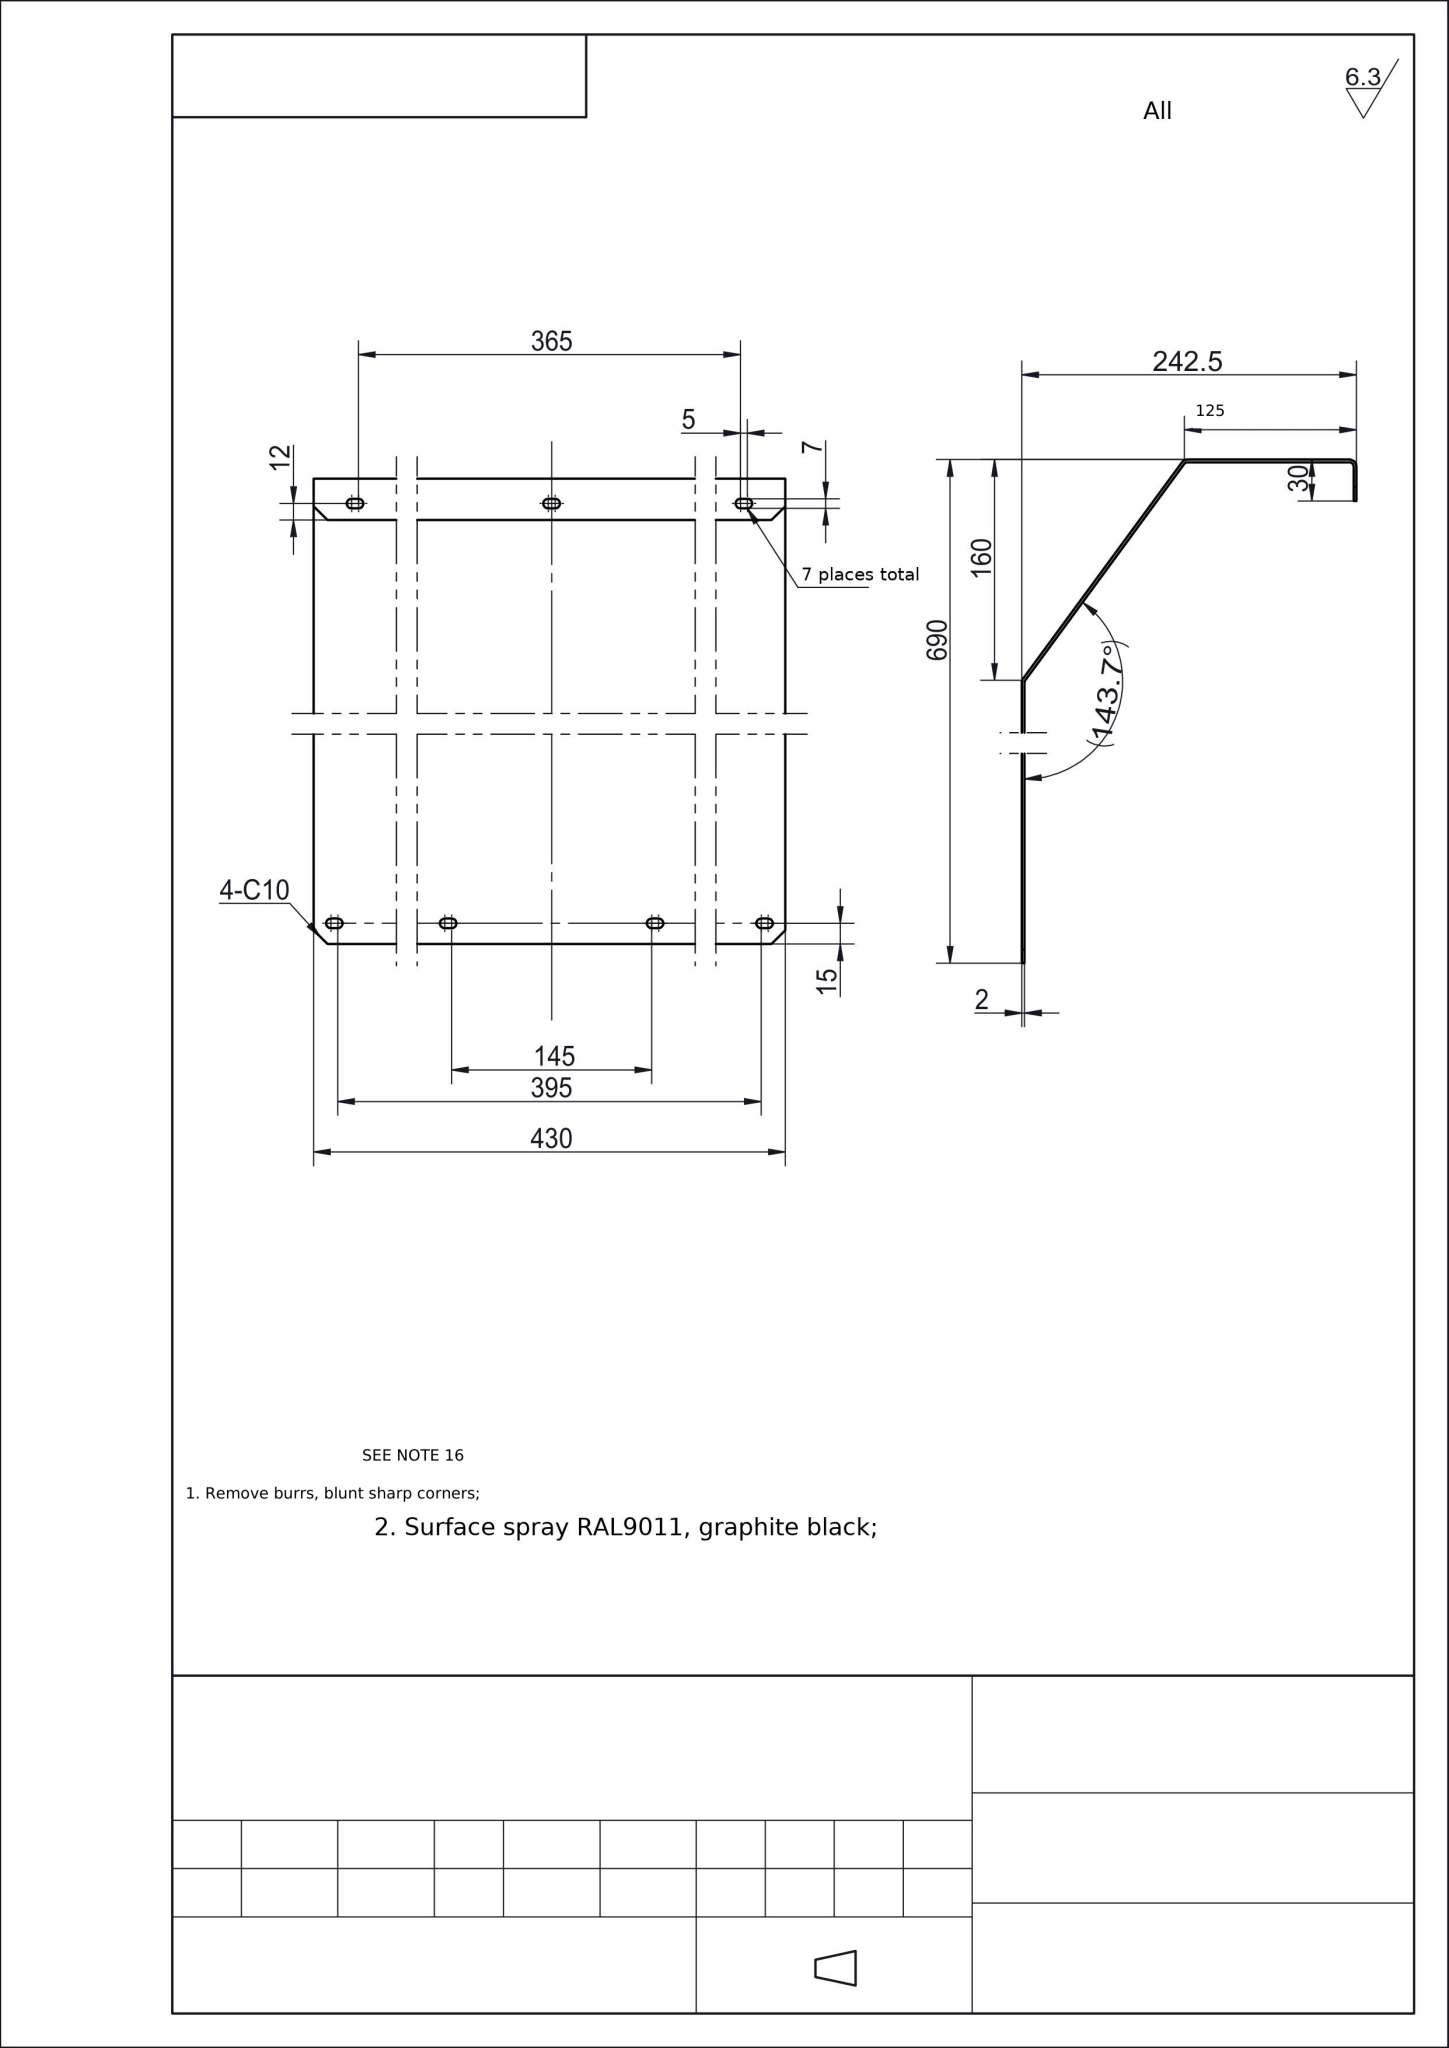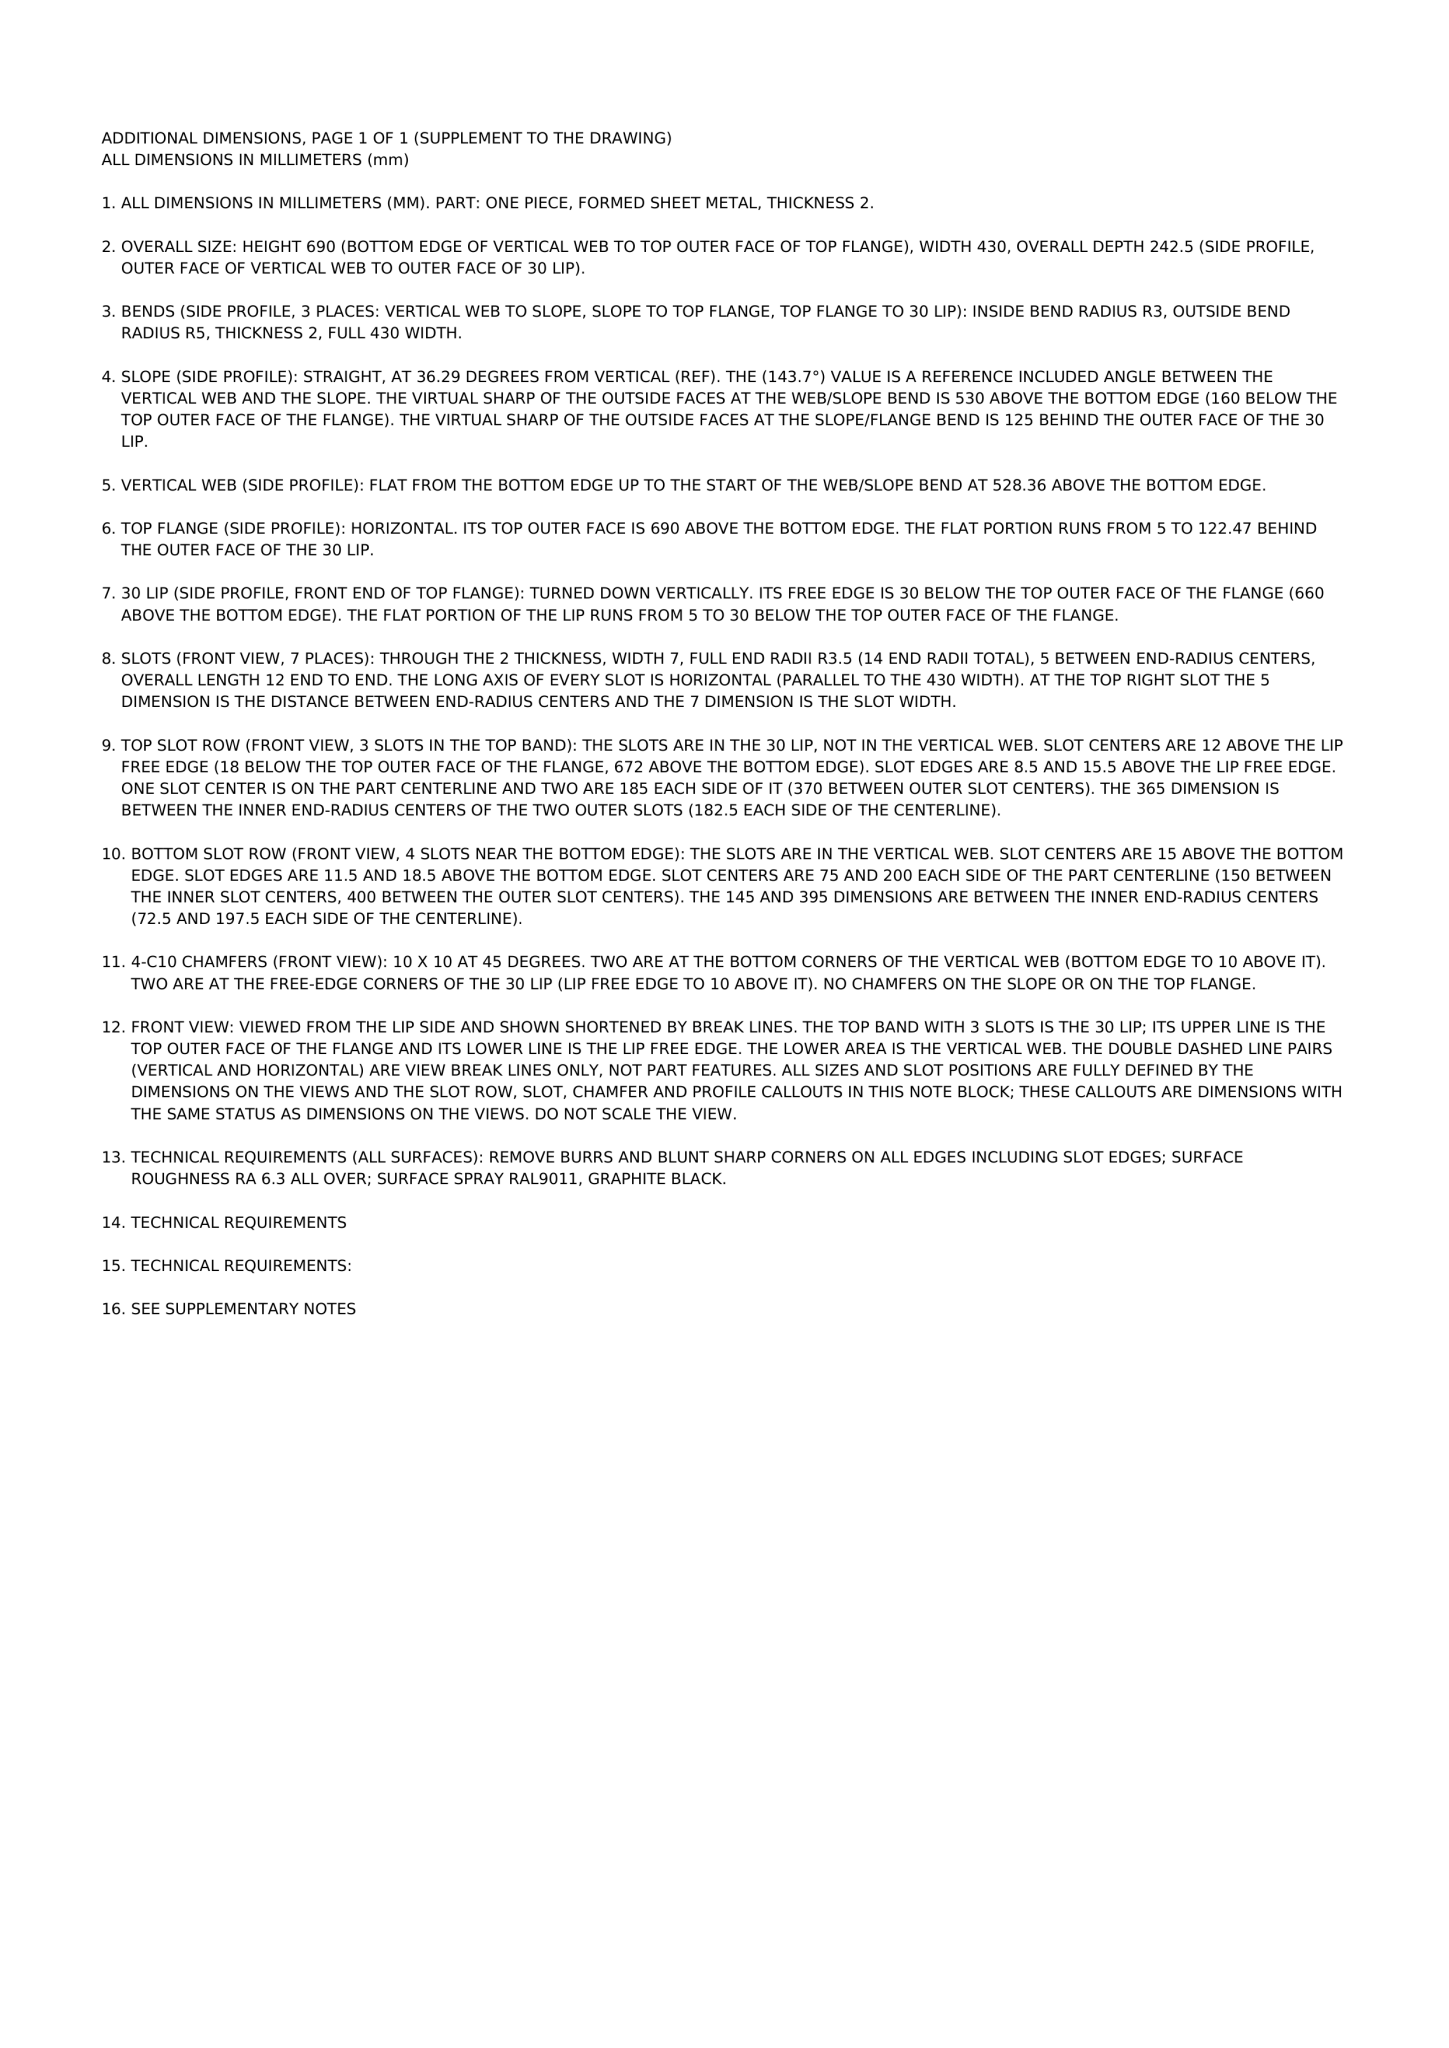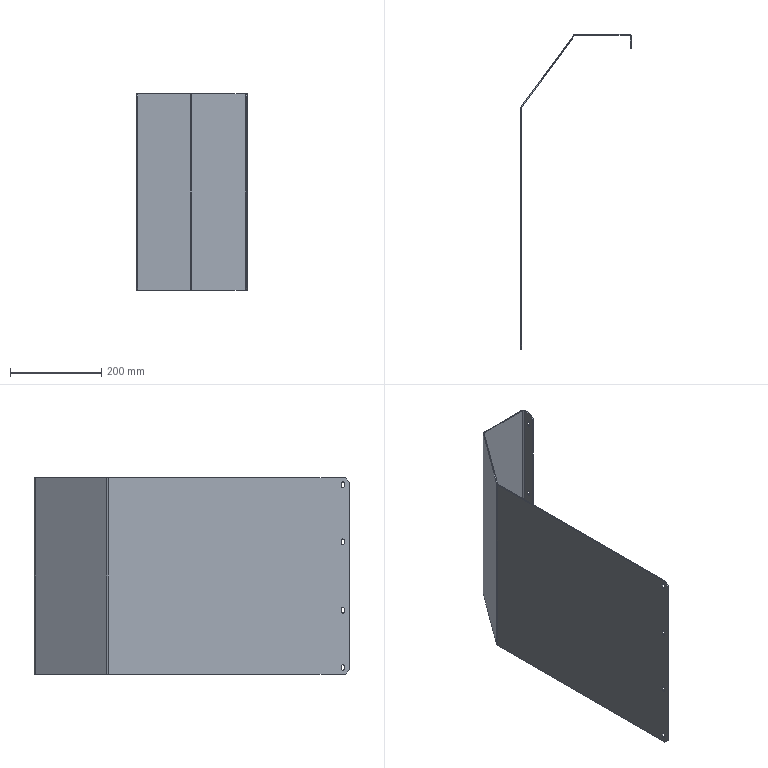Part | NX | mm | 1 solid | 66 faces | box 242.5 x 690 x 430 mm | volume 753424 mm3 | plane 42 | cylinder 24 | commonest cylinder face diameters 7 x18 10 x3 6 x3